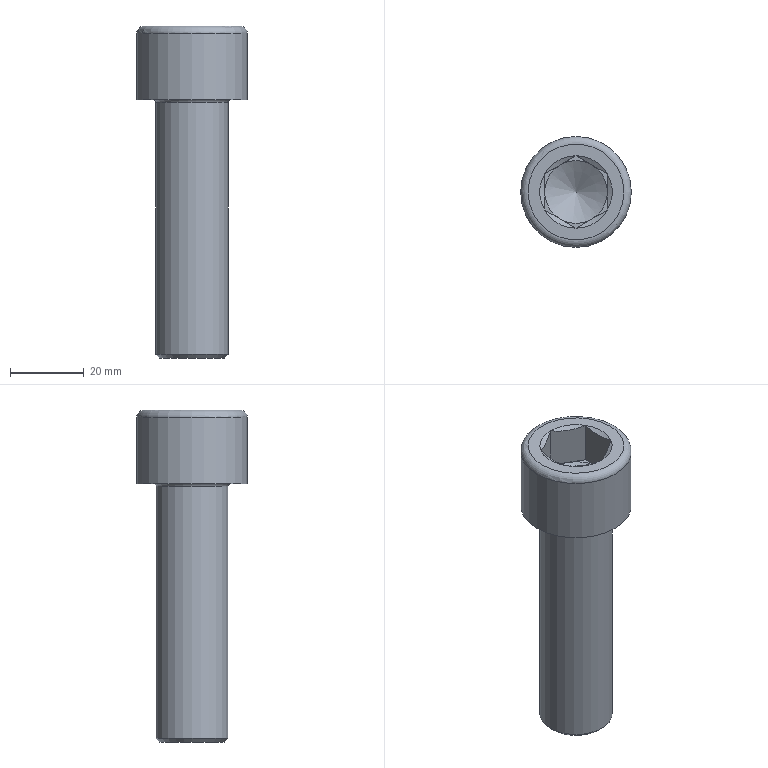Component | NX | GB-T70_1-2000_M20X70 | 1 solid | 27 faces | volume 31968 mm3 | plane 15 | cone 8 | cylinder 2 | torus 2 | commonest cylinder face diameters 19.623 x1 30 x1